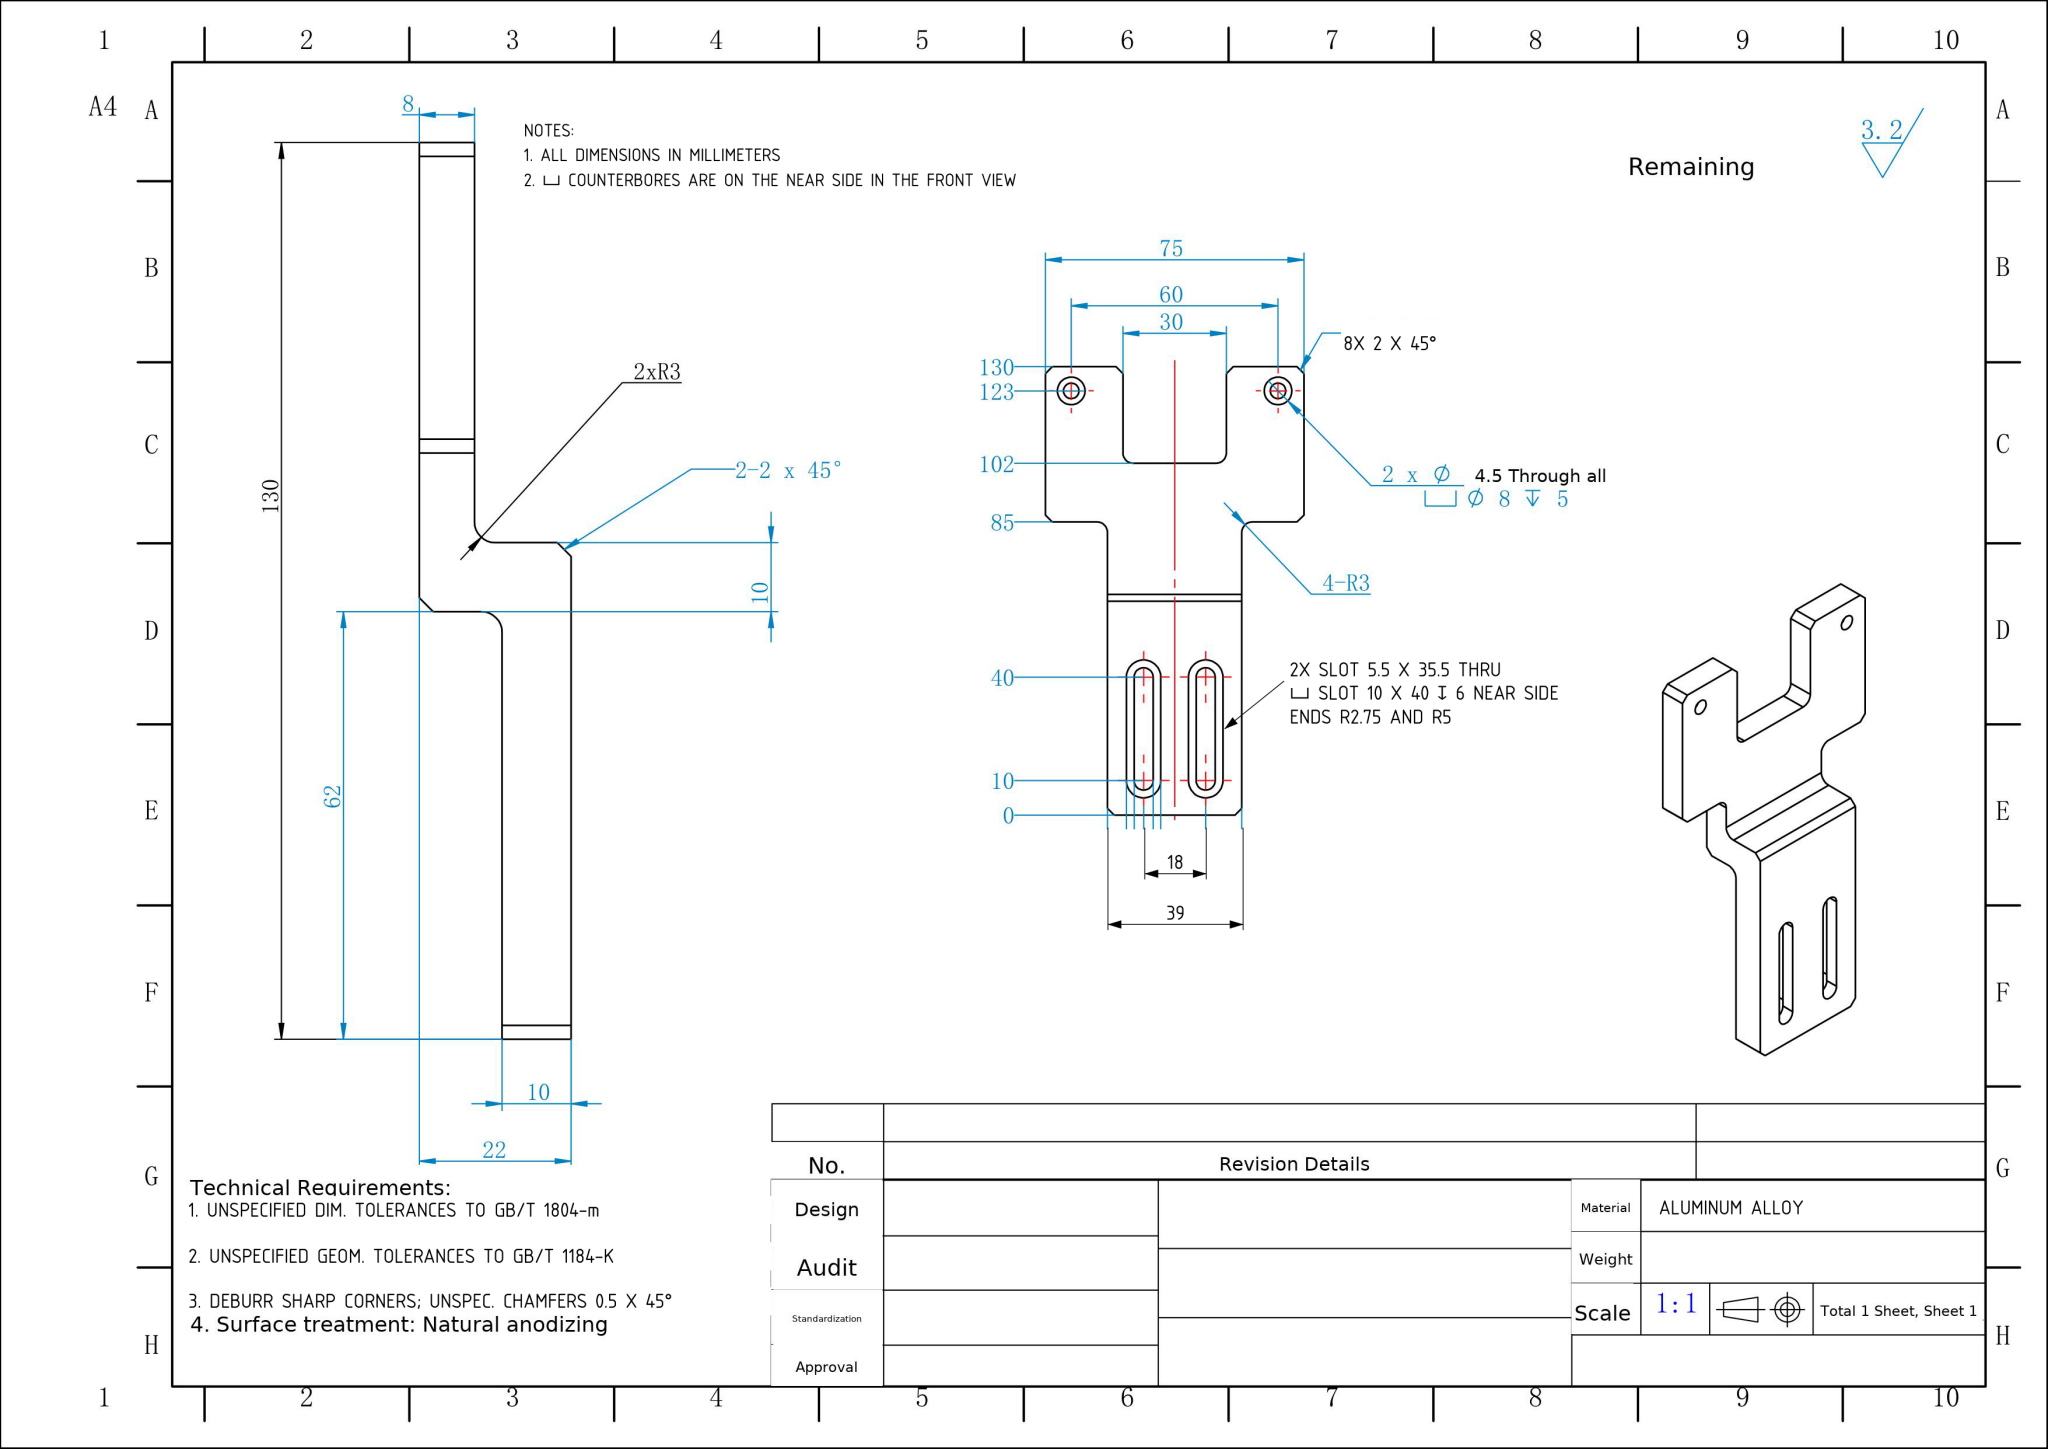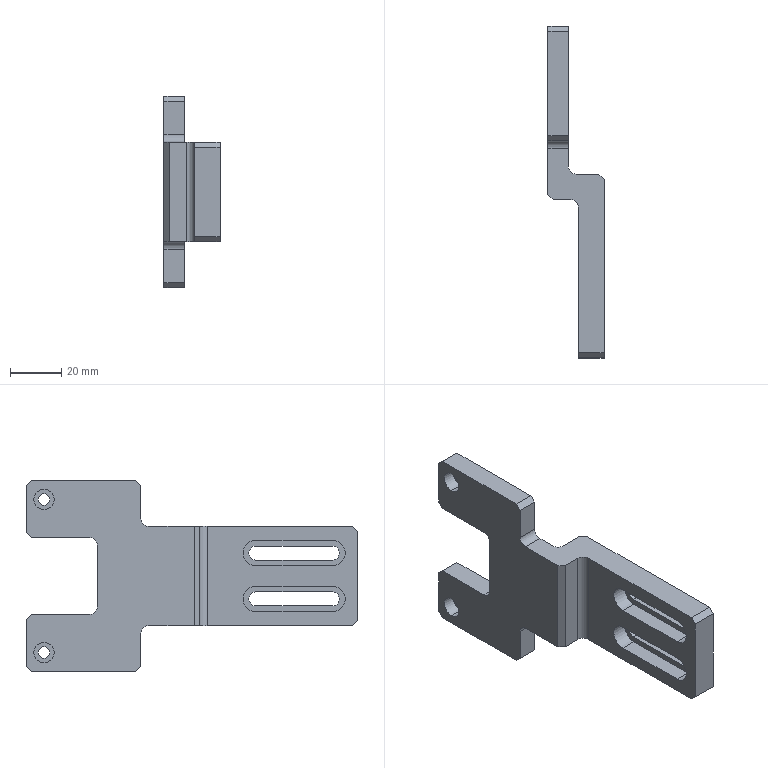Part | NX | mm | 1 solid | 62 faces | box 22 x 130 x 75 mm | volume 50366 mm3 | plane 40 | cylinder 22 | commonest cylinder face diameters 6 x6 8 x4 4.5 x4 5.5 x4 10 x4